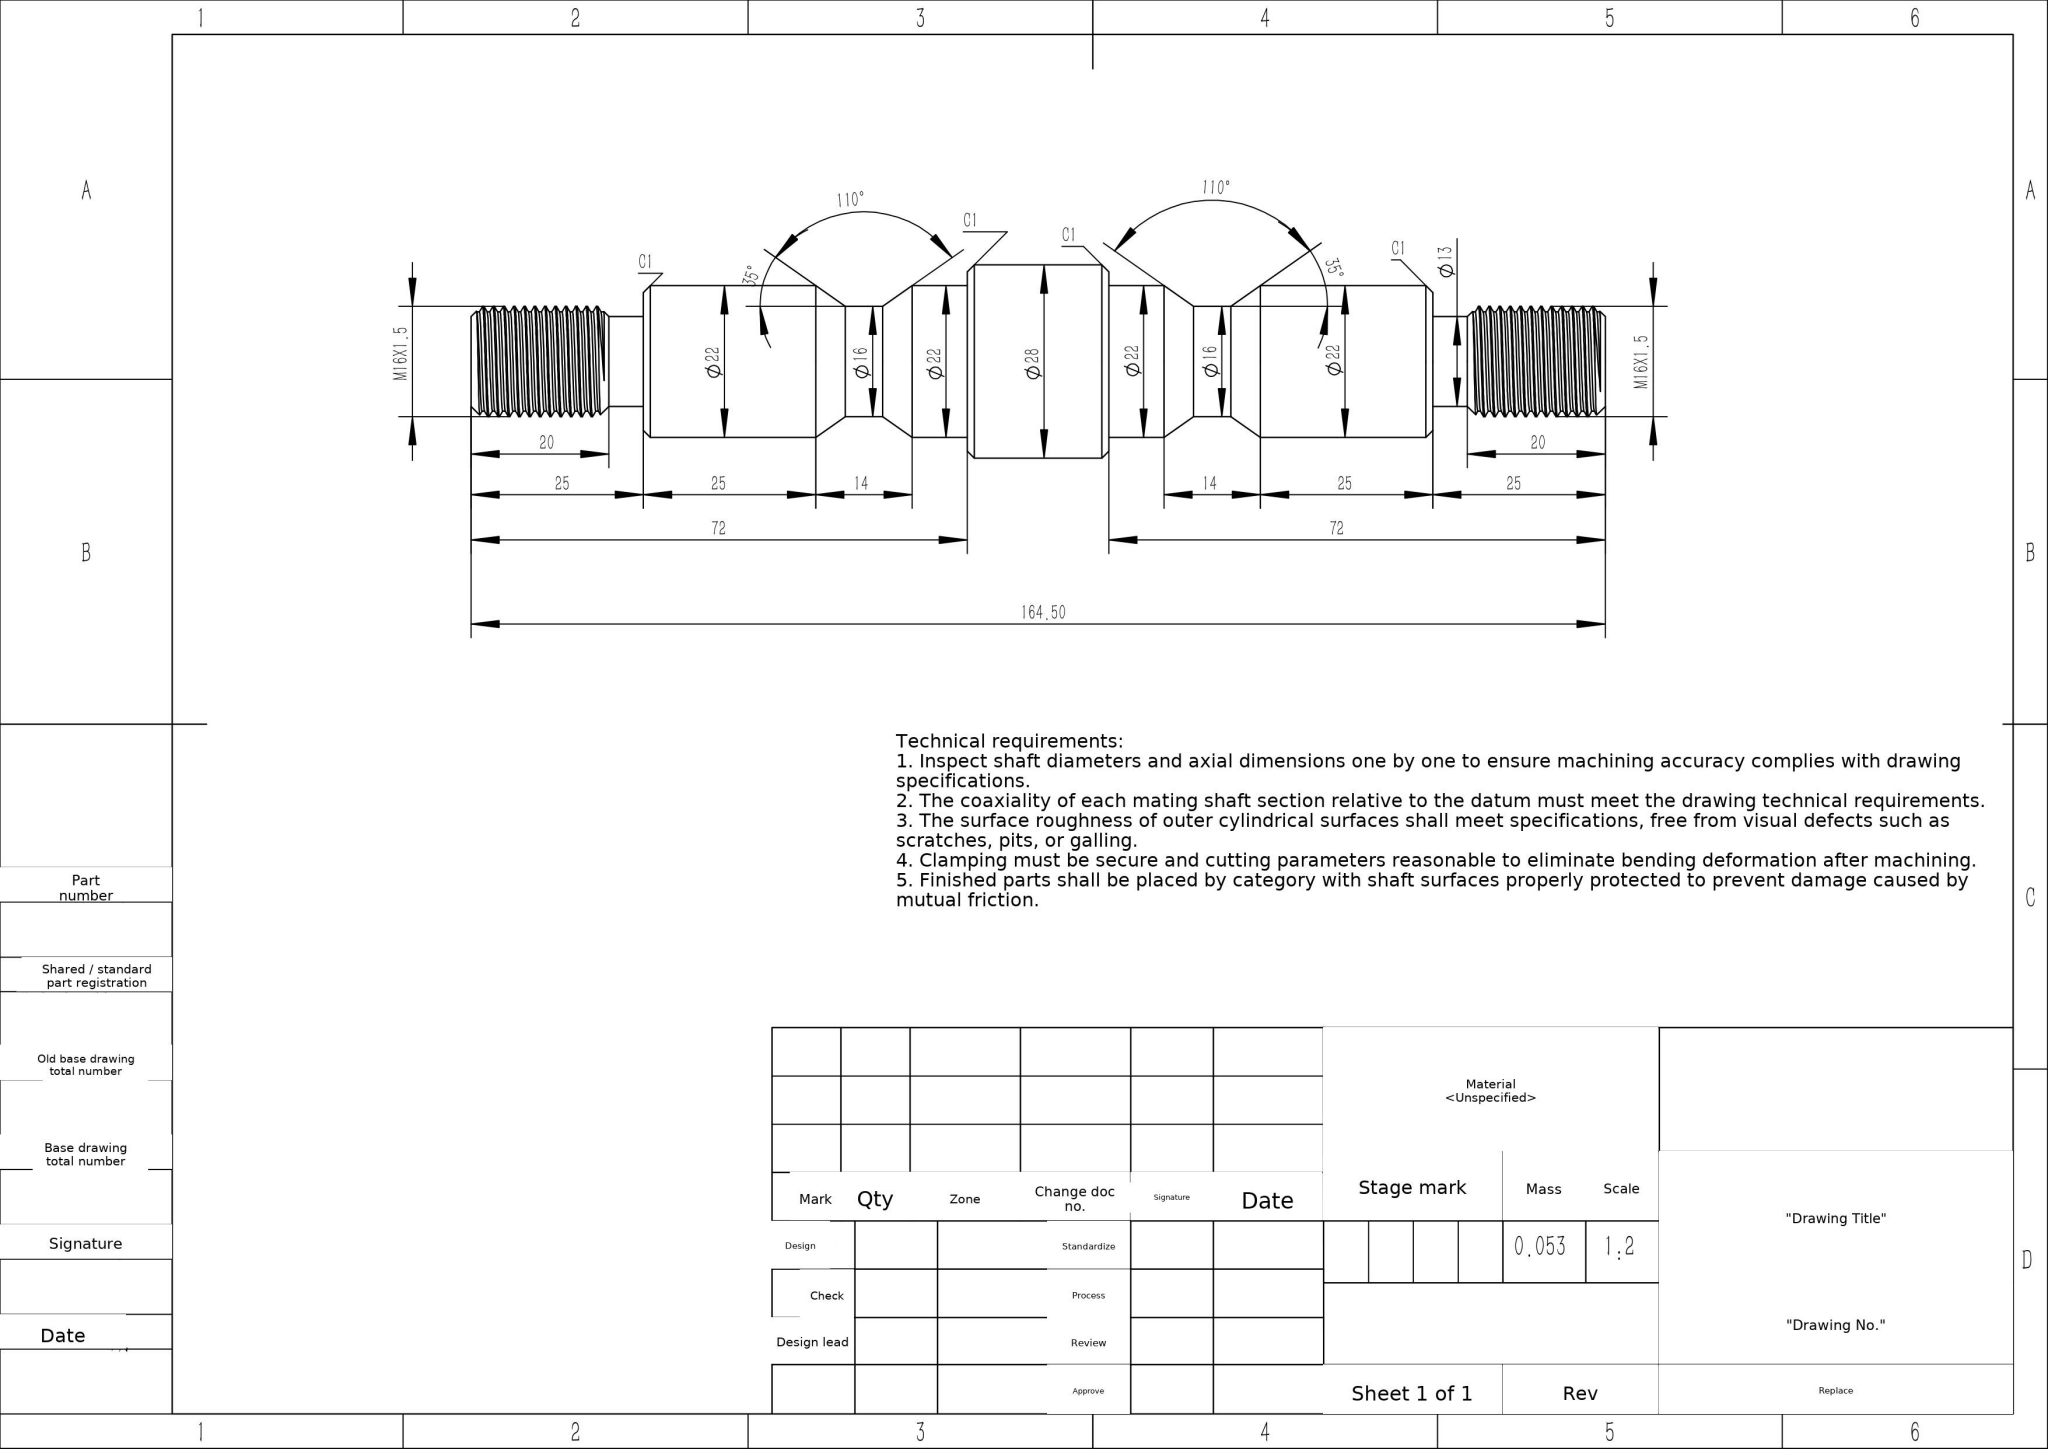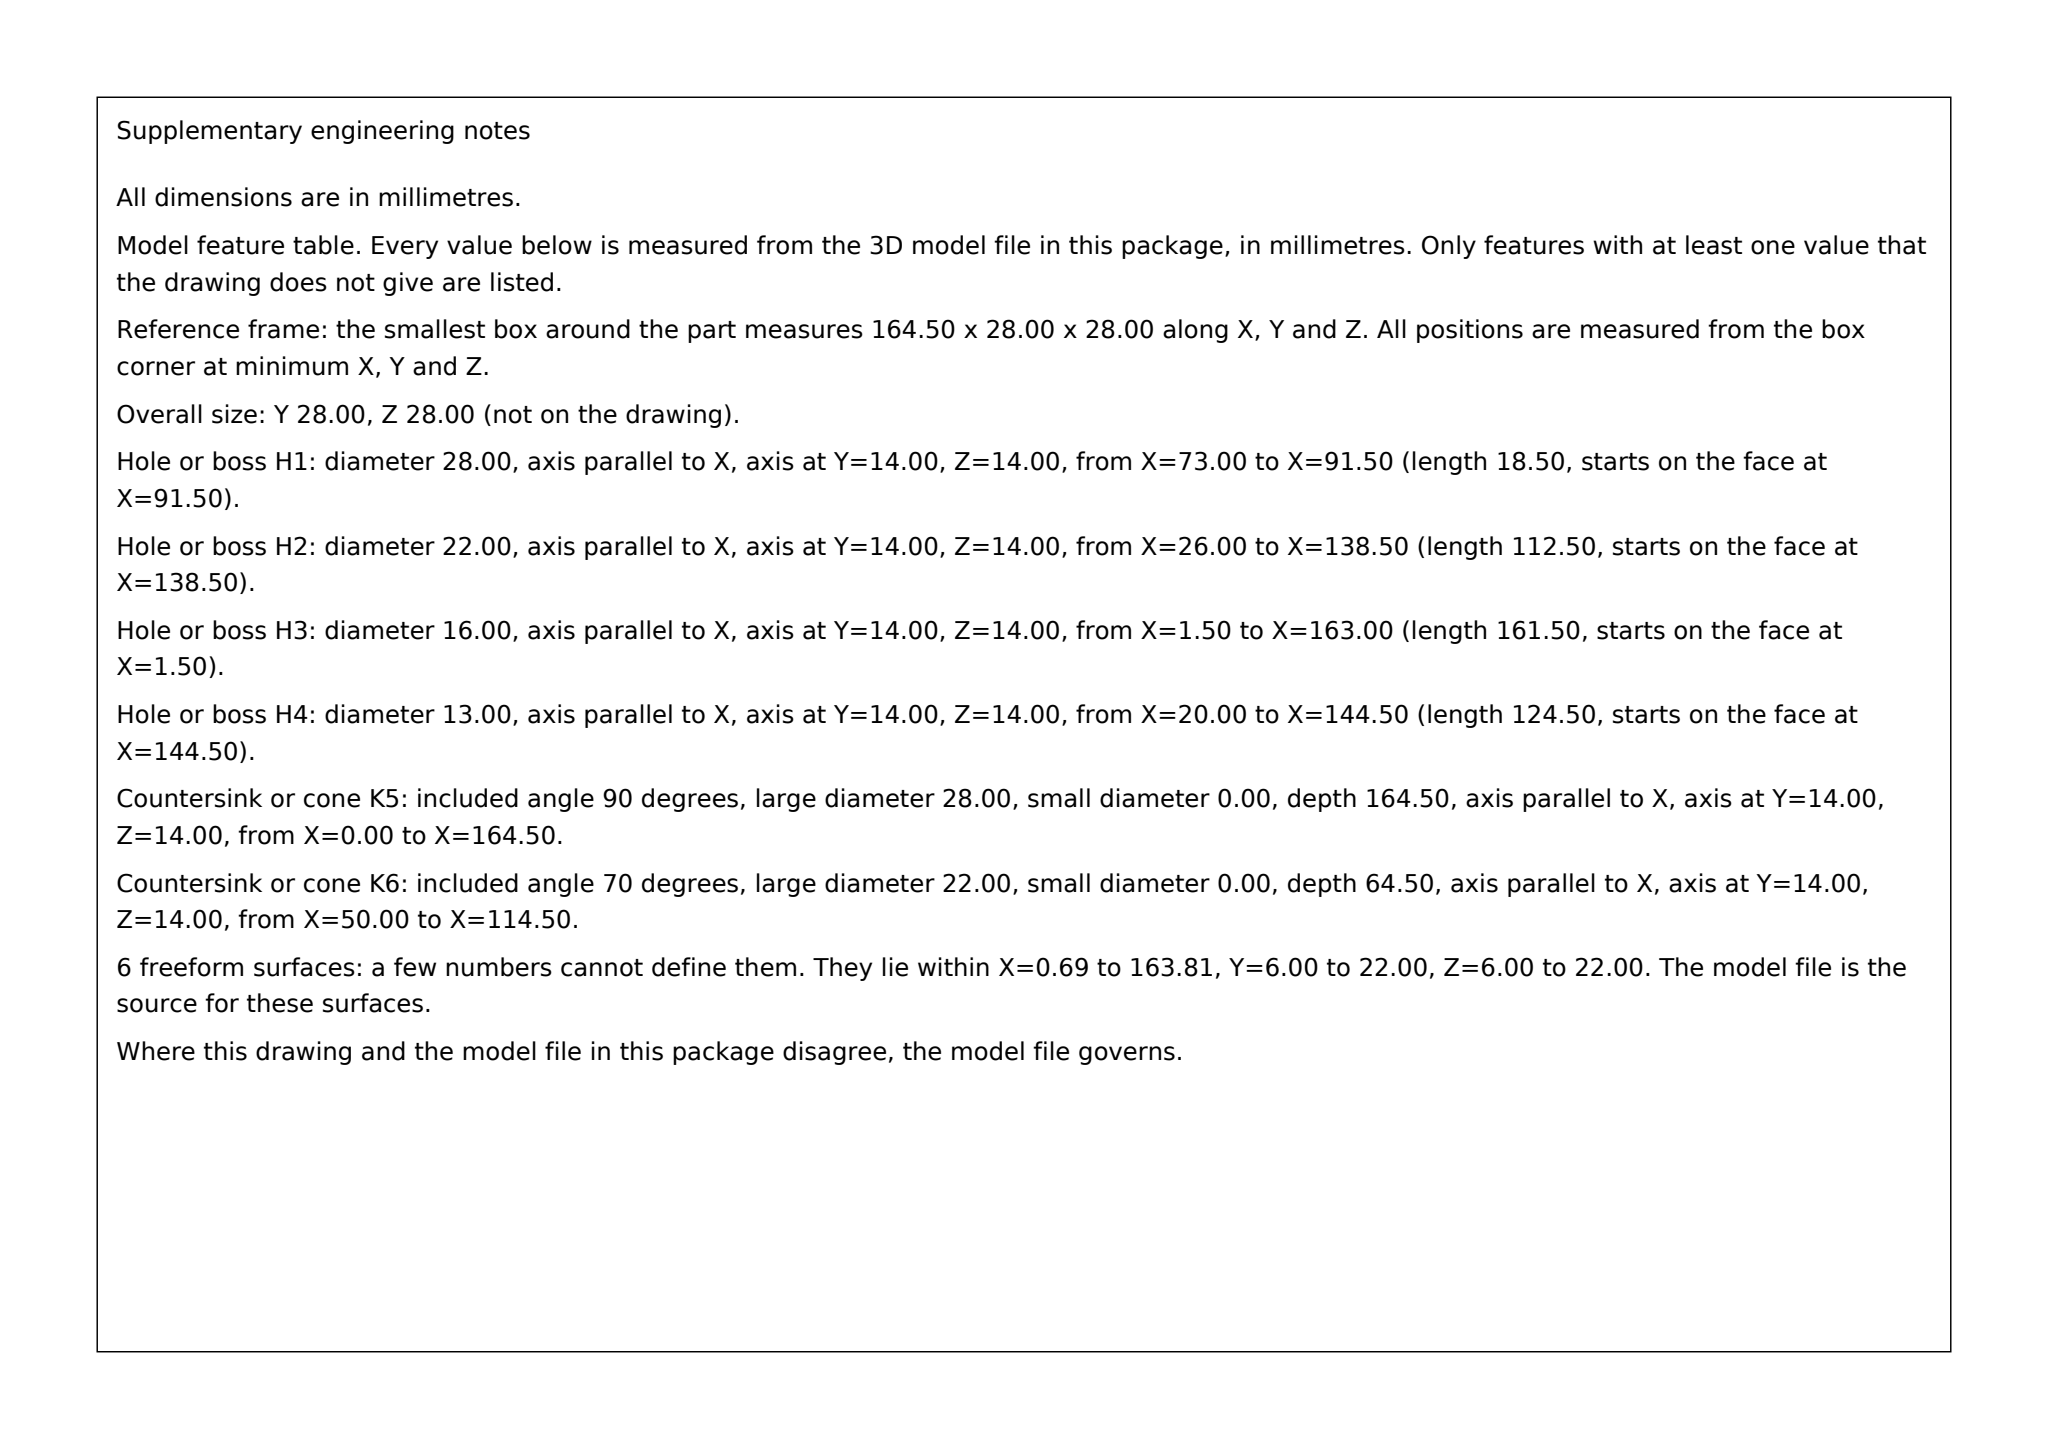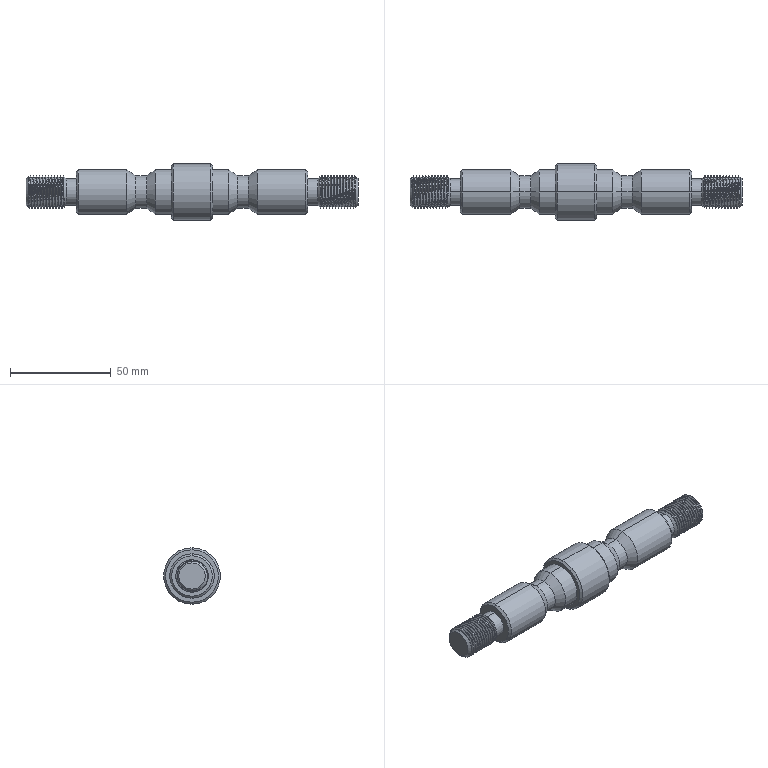Part | SolidWorks | mm | 1 solid | 104 faces | box 164.5 x 28 x 28 mm | volume 53075 mm3 | cylinder 64 | cone 28 | plane 6 | spline 6 | commonest cylinder face diameters 16 x50 22 x8 13 x4 28 x2